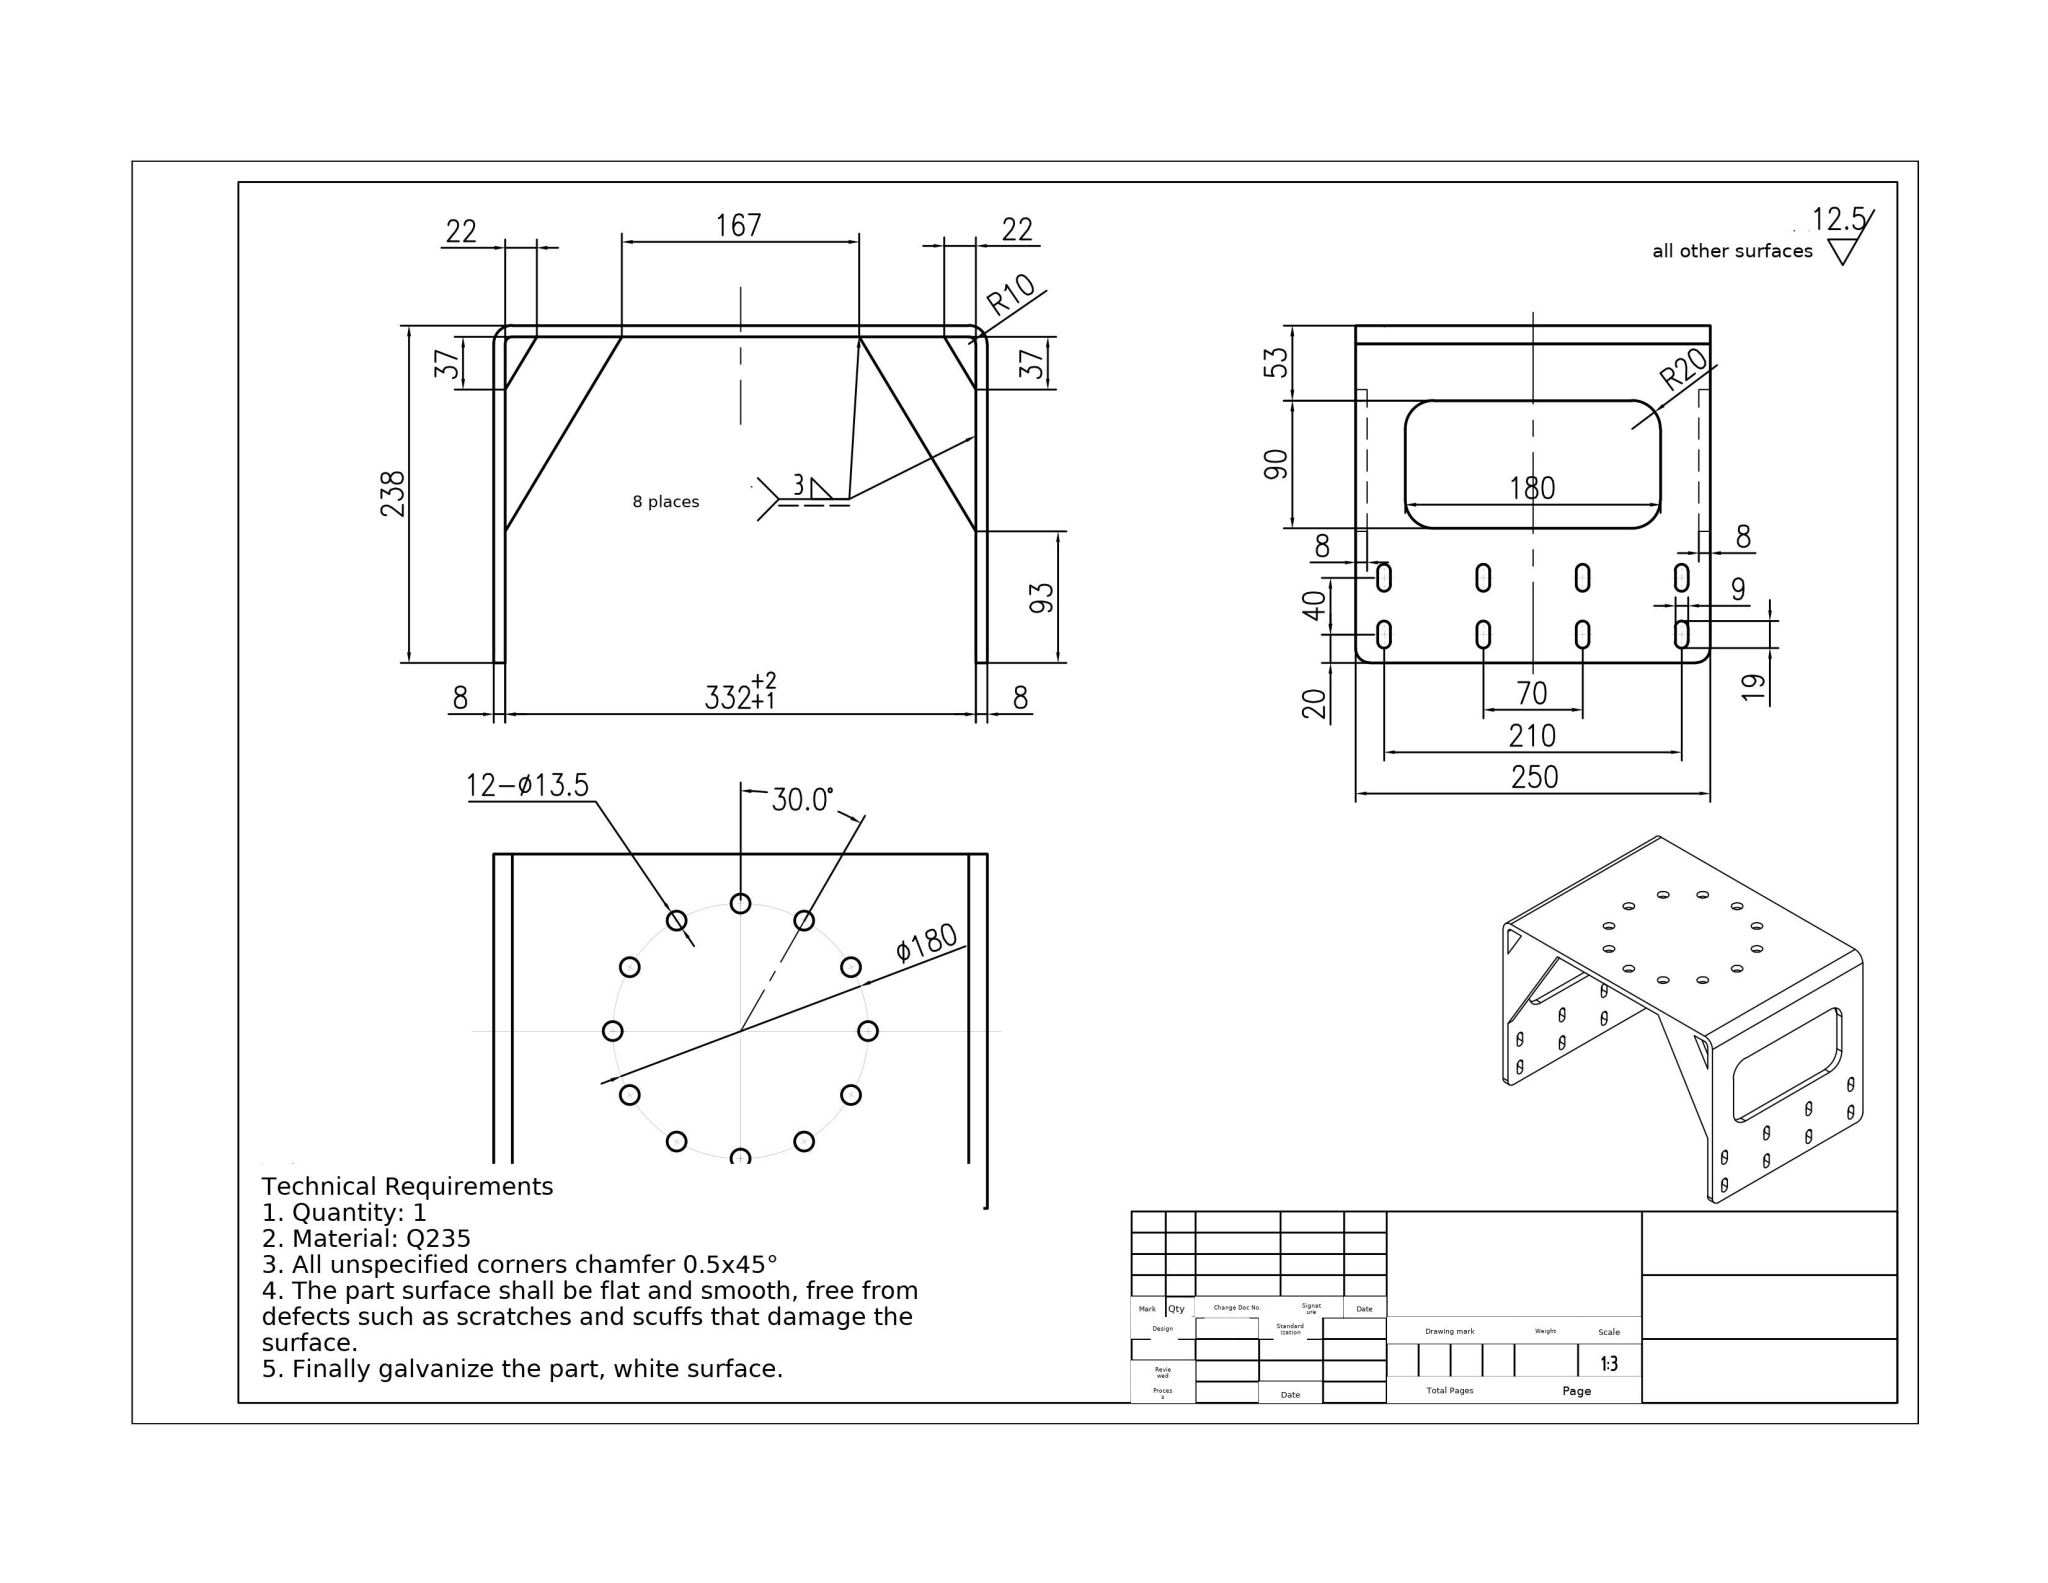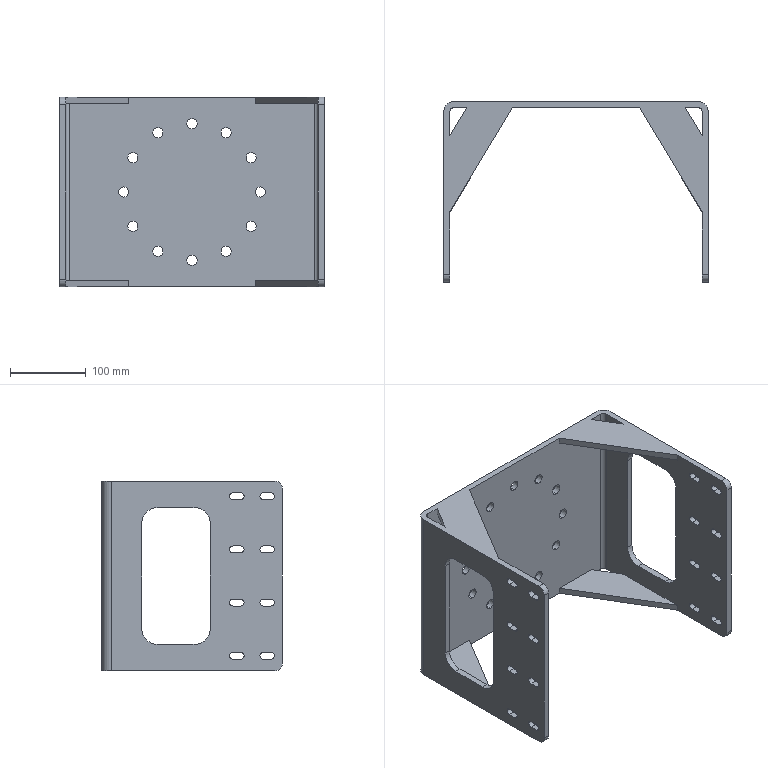Part | SolidWorks | mm | material Q235 | 1 solid | 150 faces | box 348 x 238 x 250 mm | volume 1480173 mm3 | cylinder 88 | plane 62 | commonest cylinder face diameters 9 x48 13.5 x24 40 x8 20 x4 10 x2 26 x2
build123d program:
from build123d import *

# Parameters (mm, degrees)
EXTRUDE_THIN1_DEPTH = 250
CUT_EXTRUDE3_DEPTH  = 487.317
BOSS_EXTRUDE2_DEPTH = 8
SKETCH11_W          = 180
SKETCH11_H          = 90
CUT_EXTRUDE4_DEPTH  = 487.317
FILLET1_R           = 20
FILLET2_R           = 10
CIRPATTERN1_COUNT   = 12


with BuildPart() as part:
    # Sketch2 → Extrude-Thin1 (new body)
    with BuildSketch(Plane.XY):
        with BuildLine():
            Line((-332, -230), (-332, -5))
            ThreePointArc((-332, -5), (-330.536, -1.464), (-327, 0))
            Line((-327, 0), (-5, 0))
            ThreePointArc((-5, 0), (-1.464, -1.464), (0, -5))
            Line((0, -5), (0, -230))
            Line((0, -230), (8, -230))
            Line((8, -230), (8, -5))
            ThreePointArc((8, -5), (4.192, 4.192), (-5, 8))
            Line((-5, 8), (-327, 8))
            ThreePointArc((-327, 8), (-336.192, 4.192), (-340, -5))
            Line((-340, -5), (-340, -230))
            Line((-340, -230), (-332, -230))
        make_face()
    extrude(amount=EXTRUDE_THIN1_DEPTH)

    # Sketch4 → M12 Clearance Hole1 (revolve, cut)
    with BuildSketch(Plane(origin=(-121, 8, 47.058), x_dir=(0, 0, 1), z_dir=(1, 0, 0))):
        Polygon((0, 0), (0, 19.056), (6.75, 15), (6.75, 0), align=None)
    m12_clearance_hole1 = revolve(axis=Axis((-121, 14.35, 47.058), (0, -1, 0)), mode=Mode.SUBTRACT)

    # Sketch8 → Cut-Extrude3 (cut, through all)
    with BuildSketch(Plane(origin=(8, 0, 0), x_dir=(0, 0, -1), z_dir=(1, 0, 0))):
        with BuildLine():
            Line((-225.5, -205), (-225.5, -215))
            ThreePointArc((-225.5, -215), (-230, -219.5), (-234.5, -215))
            Line((-234.5, -215), (-234.5, -205))
            ThreePointArc((-234.5, -205), (-230, -200.5), (-225.5, -205))
        make_face()
        with BuildLine():
            Line((-225.5, -165), (-225.5, -175))
            ThreePointArc((-225.5, -175), (-230, -179.5), (-234.5, -175))
            Line((-234.5, -175), (-234.5, -165))
            ThreePointArc((-234.5, -165), (-230, -160.5), (-225.5, -165))
        make_face()
        with BuildLine():
            Line((-155.5, -165), (-155.5, -175))
            ThreePointArc((-155.5, -175), (-160, -179.5), (-164.5, -175))
            Line((-164.5, -175), (-164.5, -165))
            ThreePointArc((-164.5, -165), (-160, -160.5), (-155.5, -165))
        make_face()
        with BuildLine():
            Line((-155.5, -205), (-155.5, -215))
            ThreePointArc((-155.5, -215), (-160, -219.5), (-164.5, -215))
            Line((-164.5, -215), (-164.5, -205))
            ThreePointArc((-164.5, -205), (-160, -200.5), (-155.5, -205))
        make_face()
        with BuildLine():
            Line((-94.5, -205), (-94.5, -215))
            ThreePointArc((-94.5, -215), (-90, -219.5), (-85.5, -215))
            Line((-85.5, -215), (-85.5, -205))
            ThreePointArc((-85.5, -205), (-90, -200.5), (-94.5, -205))
        make_face()
        with BuildLine():
            Line((-94.5, -165), (-94.5, -175))
            ThreePointArc((-94.5, -175), (-90, -179.5), (-85.5, -175))
            Line((-85.5, -175), (-85.5, -165))
            ThreePointArc((-85.5, -165), (-90, -160.5), (-94.5, -165))
        make_face()
        with BuildLine():
            Line((-24.5, -165), (-24.5, -175))
            ThreePointArc((-24.5, -175), (-20, -179.5), (-15.5, -175))
            Line((-15.5, -175), (-15.5, -165))
            ThreePointArc((-15.5, -165), (-20, -160.5), (-24.5, -165))
        make_face()
        with BuildLine():
            Line((-24.5, -205), (-24.5, -215))
            ThreePointArc((-24.5, -215), (-20, -219.5), (-15.5, -215))
            Line((-15.5, -215), (-15.5, -205))
            ThreePointArc((-15.5, -205), (-20, -200.5), (-24.5, -205))
        make_face()
    extrude(amount=-CUT_EXTRUDE3_DEPTH, mode=Mode.SUBTRACT)

    # Sketch10 → Boss-Extrude2 (add)
    with BuildSketch(Plane.XY.offset(250)):
        Polygon((-249.681, 0), (-332, -137.199), (-332, -37.199), (-309.681, 0), align=None)
        Polygon((-22.319, 0), (-82.319, 0), (0, -137.199), (0, -37.199), align=None)
    boss_extrude2 = extrude(amount=-BOSS_EXTRUDE2_DEPTH)

    # Mirror4: Boss-Extrude2 across plane
    add(boss_extrude2.mirror(Plane.XY.offset(125)))

    # Sketch11 → Cut-Extrude4 (cut, through all)
    with BuildSketch(Plane(origin=(8, 0, 0), x_dir=(0, 0, -1), z_dir=(1, 0, 0))):
        with Locations((-125, -90)):
            Rectangle(SKETCH11_W, SKETCH11_H)
    extrude(amount=-CUT_EXTRUDE4_DEPTH, mode=Mode.SUBTRACT)

    # Fillet1
    fillet1_edges = [part.edges().sort_by_distance(p)[0] for p in [
        (4, -45, 35),
        (4, -135, 35),
        (4, -135, 215),
        (4, -45, 215),
        (-336, -45, 35),
        (-336, -135, 35),
        (-336, -135, 215),
        (-336, -45, 215),
    ]]
    fillet(fillet1_edges, radius=FILLET1_R)

    # Fillet2
    fillet2_edges = [part.edges().sort_by_distance(p)[0] for p in [
        (4, -230, 0),
        (-336, -230, 0),
        (4, -230, 250),
        (-336, -230, 250),
    ]]
    fillet(fillet2_edges, radius=FILLET2_R)

    # CirPattern1: M12 Clearance Hole1 ×12 about axis
    cirpattern1_axis = Axis((-166, 0, 125), (0, 1, 0))
    for i in range(1, CIRPATTERN1_COUNT):
        add(m12_clearance_hole1.rotate(cirpattern1_axis, i * 360 / CIRPATTERN1_COUNT), mode=Mode.SUBTRACT)


solid = part.part